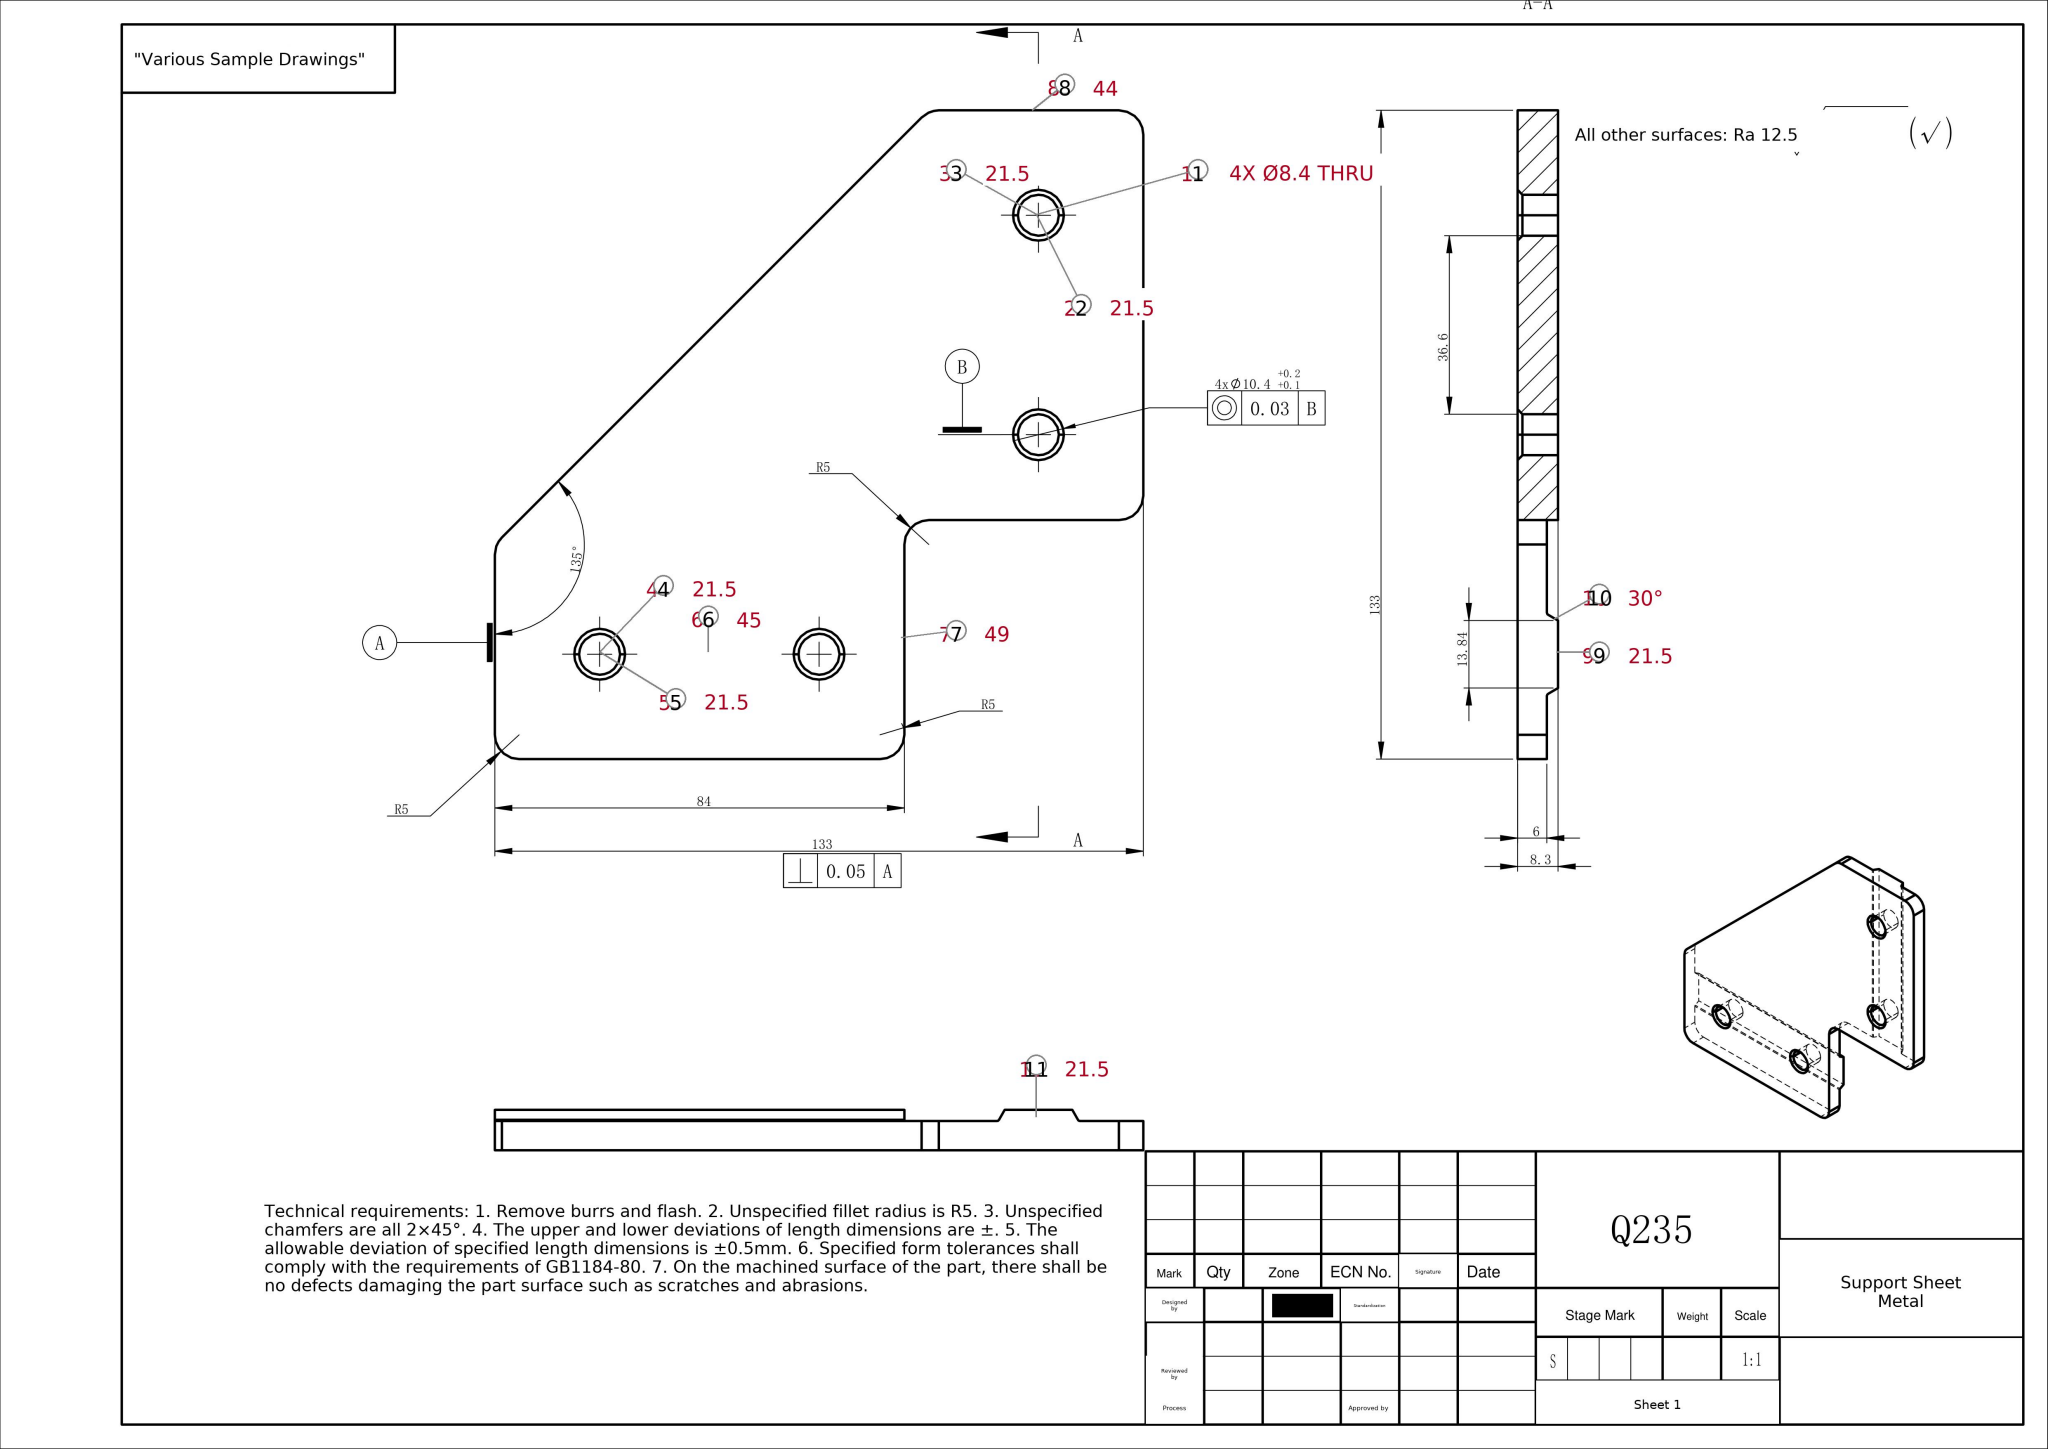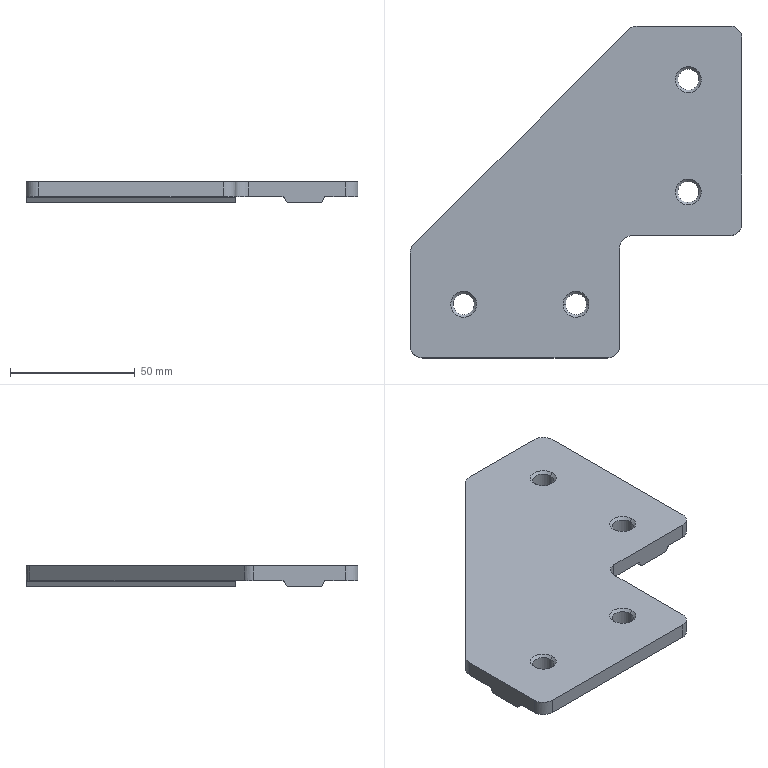Part | SolidWorks | mm | material Q235 | 1 solid | 44 faces | box 133 x 133 x 8.3 mm | volume 71833 mm3 | spline 44